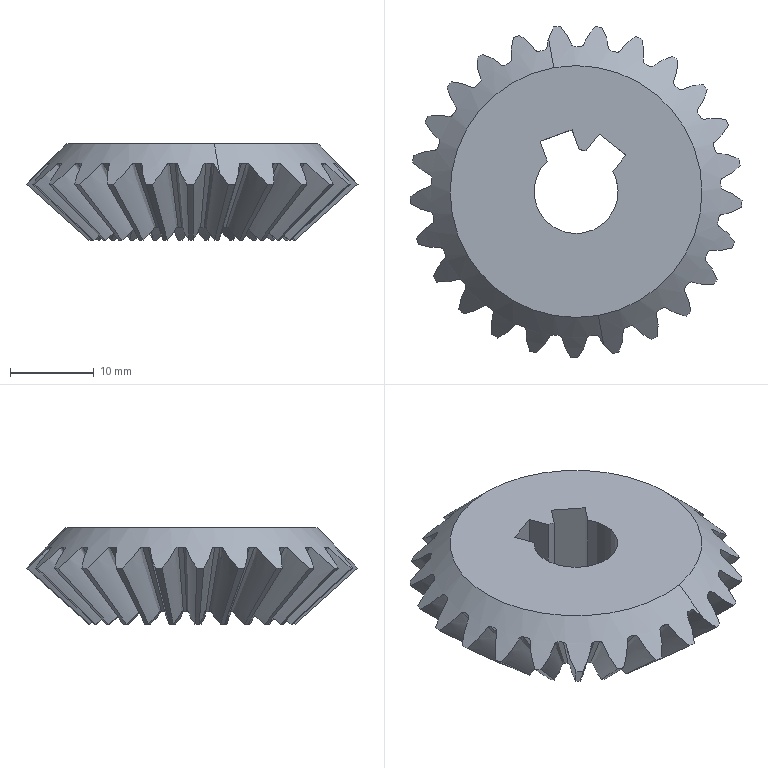Component | SolidWorks | NormalGear-1 | 1 solid | 139 faces | volume 7055 mm3 | cone 53 | spline 50 | plane 33 | cylinder 3 | commonest cylinder face diameters 10.015 x3